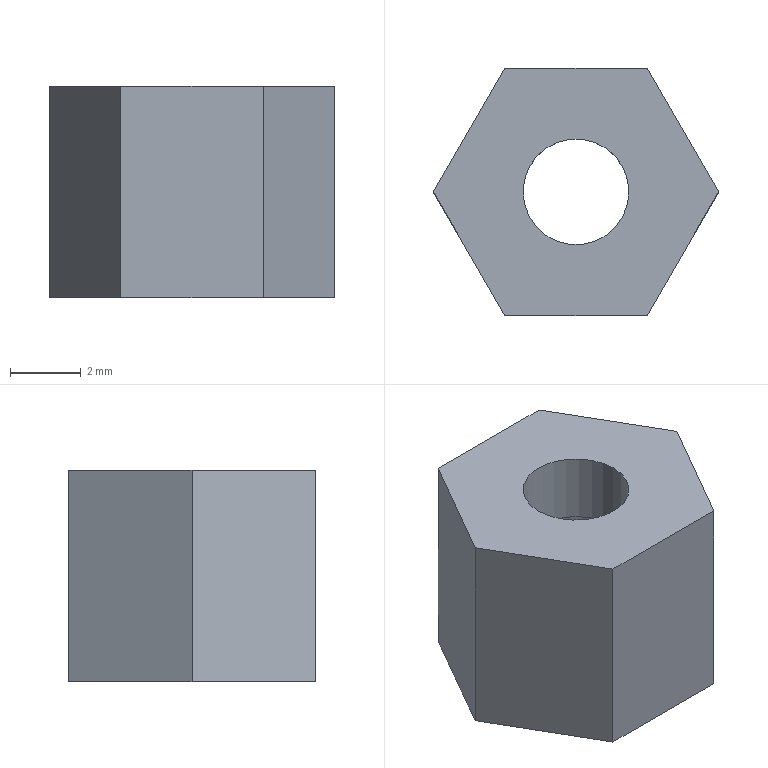Component | NX | EXT_PIPE_CONN_BLOCK | 1 solid | 11 faces | volume 127 mm3 | plane 9 | cylinder 2 | commonest cylinder face diameters 6 x1 3 x1